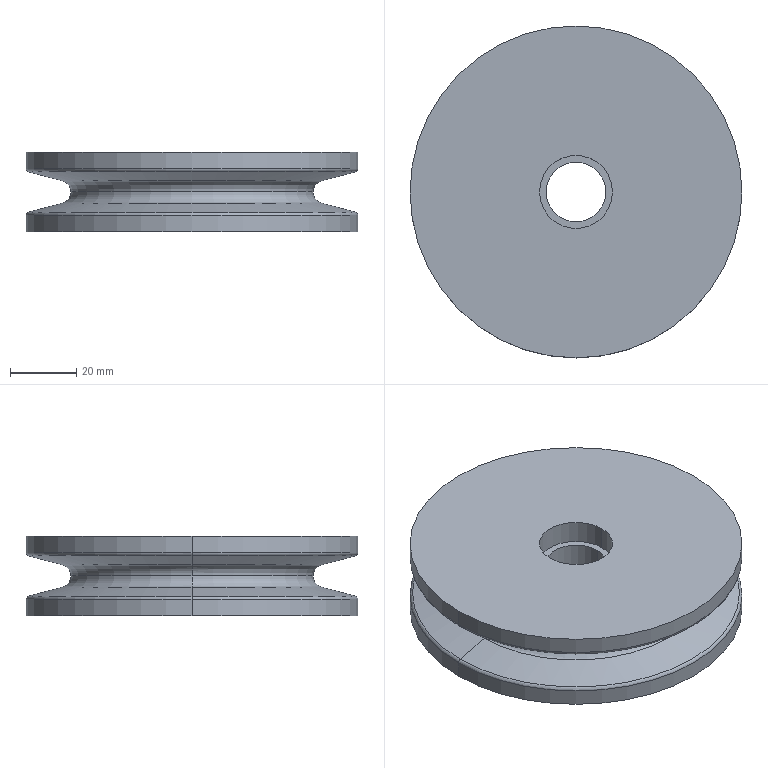Component | SolidWorks | JL001-05-02-1_JL001-05-01-004-2 | 1 solid | 26 faces | box 100 x 100 x 24 mm | volume 147536 mm3 | cylinder 10 | torus 8 | cone 4 | plane 4 | commonest cylinder face diameters 22 x4 100 x4 18 x2
build123d program:
from build123d import *

# Parameters (mm, degrees)
FILLET1_R = 1


with BuildPart() as part:
    # Sketch1 → Revolve1 (revolve)
    with BuildSketch(Plane.XY, mode=Mode.PRIVATE) as revolve1_sk:
        Polygon((11, 12), (50, 12), (50, -12), (11, -12), (11, -5), (9, -5), (9, 5), (11, 5), align=None)
    revolve(revolve1_sk.sketch.rotate(Axis((0, 0, 0), (0, -1, 0)), 90), axis=Axis((0, 0, 0), (0, -1, 0)))

    # Sketch2 → Cut-Revolve1 (revolve, cut)
    with BuildSketch(Plane.XY, mode=Mode.PRIVATE) as cut_revolve1_sk:
        with BuildLine():
            Line((39.094, 3.381), (51, 6.571))
            Line((51, 6.571), (51, -6.571))
            Line((51, -6.571), (39.094, -3.381))
            ThreePointArc((39.094, -3.381), (36.5, 0), (39.094, 3.381))
        make_face()
    revolve(cut_revolve1_sk.sketch.rotate(Axis((0, 0, 0), (0, -1, 0)), 90), axis=Axis((0, 0, 0), (0, -1, 0)), mode=Mode.SUBTRACT)

    # Fillet1
    fillet1_edges = [part.edges().sort_by_distance(p)[0] for p in [
        (0, -6.303, -50),
        (0, 6.303, -50),
    ]]
    fillet(fillet1_edges, radius=FILLET1_R)


solid = part.part

# Placed as in the assembly
solid = solid.moved(Location((0, 1047.5, 76), (90, 0, 0)))
STEP:
#1=COLOUR_RGB('',0.7922,0.8196,0.9333);
#2=FILL_AREA_STYLE_COLOUR('',#1);
#3=FILL_AREA_STYLE('',(#2));
#4=SURFACE_STYLE_FILL_AREA(#3);
#5=SURFACE_SIDE_STYLE('',(#4));
#6=SURFACE_STYLE_USAGE(.BOTH.,#5);
#7=PRESENTATION_STYLE_ASSIGNMENT((#6));
#8=CARTESIAN_POINT('',(-1.539,41.24,2.859));
#9=VERTEX_POINT('',#8);
#10=CARTESIAN_POINT('',(-1.437,41.24,2.992));
#11=VERTEX_POINT('',#10);
#12=CARTESIAN_POINT('',(-1.575,41.24,2.992));
#13=DIRECTION('',(0.,-1.,0.));
#14=DIRECTION('',(0.,0.,-1.));
#15=AXIS2_PLACEMENT_3D('',#12,#13,#14);
#16=CIRCLE('',#15,0.1378);
#17=EDGE_CURVE('',#9,#11,#16,.T.);
#18=ORIENTED_EDGE('',*,*,#17,.T.);
#19=CARTESIAN_POINT('',(1.437,41.24,2.992));
#20=VERTEX_POINT('',#19);
#21=CARTESIAN_POINT('',(-0.,41.24,2.992));
#22=DIRECTION('',(-0.,-0.,-1.));
#23=DIRECTION('',(0.,1.,0.));
#24=AXIS2_PLACEMENT_3D('',#21,#22,#23);
#25=CIRCLE('',#24,1.437);
#26=EDGE_CURVE('',#11,#20,#25,.T.);
#27=ORIENTED_EDGE('',*,*,#26,.T.);
#28=CARTESIAN_POINT('',(1.539,41.24,2.859));
#29=VERTEX_POINT('',#28);
#30=CARTESIAN_POINT('',(1.575,41.24,2.992));
#31=DIRECTION('',(-0.,1.,-0.));
#32=DIRECTION('',(0.,0.,1.));
#33=AXIS2_PLACEMENT_3D('',#30,#31,#32);
#34=CIRCLE('',#33,0.1378);
#35=EDGE_CURVE('',#29,#20,#34,.T.);
#36=ORIENTED_EDGE('',*,*,#35,.F.);
#37=CARTESIAN_POINT('',(-0.,41.24,2.859));
#38=DIRECTION('',(-0.,-0.,-1.));
#39=DIRECTION('',(-1.,0.,0.));
#40=AXIS2_PLACEMENT_3D('',#37,#38,#39);
#41=CIRCLE('',#40,1.539);
#42=EDGE_CURVE('',#9,#29,#41,.T.);
#43=ORIENTED_EDGE('',*,*,#42,.F.);
#44=EDGE_LOOP('',(#18,#27,#36,#43));
#45=FACE_OUTER_BOUND('',#44,.T.);
#46=CARTESIAN_POINT('',(-0.,41.24,2.992));
#47=DIRECTION('',(-0.,-0.,-1.));
#48=DIRECTION('',(-1.,0.,0.));
#49=AXIS2_PLACEMENT_3D('',#46,#47,#48);
#50=TOROIDAL_SURFACE('',#49,1.575,0.1378);
#51=ADVANCED_FACE('',(#45),#50,.F.);
#52=ORIENTED_EDGE('',*,*,#35,.T.);
#53=CARTESIAN_POINT('',(-0.,41.24,2.992));
#54=DIRECTION('',(-0.,-0.,-1.));
#55=DIRECTION('',(0.,1.,0.));
#56=AXIS2_PLACEMENT_3D('',#53,#54,#55);
#57=CIRCLE('',#56,1.437);
#58=EDGE_CURVE('',#20,#11,#57,.T.);
#59=ORIENTED_EDGE('',*,*,#58,.T.);
#60=ORIENTED_EDGE('',*,*,#17,.F.);
#61=CARTESIAN_POINT('',(-0.,41.24,2.859));
#62=DIRECTION('',(-0.,-0.,-1.));
#63=DIRECTION('',(-1.,0.,0.));
#64=AXIS2_PLACEMENT_3D('',#61,#62,#63);
#65=CIRCLE('',#64,1.539);
#66=EDGE_CURVE('',#29,#9,#65,.T.);
#67=ORIENTED_EDGE('',*,*,#66,.F.);
#68=EDGE_LOOP('',(#52,#59,#60,#67));
#69=FACE_OUTER_BOUND('',#68,.T.);
#70=CARTESIAN_POINT('',(-0.,41.24,2.992));
#71=DIRECTION('',(-0.,-0.,-1.));
#72=DIRECTION('',(-1.,0.,0.));
#73=AXIS2_PLACEMENT_3D('',#70,#71,#72);
#74=TOROIDAL_SURFACE('',#73,1.575,0.1378);
#75=ADVANCED_FACE('',(#69),#74,.F.);
#76=CARTESIAN_POINT('',(1.939,41.24,2.752));
#77=VERTEX_POINT('',#76);
#78=CARTESIAN_POINT('',(-1.939,41.24,2.752));
#79=VERTEX_POINT('',#78);
#80=CARTESIAN_POINT('',(-0.,41.24,2.752));
#81=DIRECTION('',(0.,0.,1.));
#82=DIRECTION('',(-1.,0.,0.));
#83=AXIS2_PLACEMENT_3D('',#80,#81,#82);
#84=CIRCLE('',#83,1.939);
#85=EDGE_CURVE('',#77,#79,#84,.T.);
#86=ORIENTED_EDGE('',*,*,#85,.F.);
#87=CARTESIAN_POINT('',(1.969,41.24,2.714));
#88=VERTEX_POINT('',#87);
#89=CARTESIAN_POINT('',(1.929,41.24,2.714));
#90=DIRECTION('',(-0.,1.,-0.));
#91=DIRECTION('',(0.,0.,1.));
#92=AXIS2_PLACEMENT_3D('',#89,#90,#91);
#93=CIRCLE('',#92,0.03937);
#94=EDGE_CURVE('',#77,#88,#93,.T.);
#95=ORIENTED_EDGE('',*,*,#94,.T.);
#96=CARTESIAN_POINT('',(-1.969,41.24,2.714));
#97=VERTEX_POINT('',#96);
#98=CARTESIAN_POINT('',(-0.,41.24,2.714));
#99=DIRECTION('',(-0.,-0.,-1.));
#100=DIRECTION('',(-1.,0.,0.));
#101=AXIS2_PLACEMENT_3D('',#98,#99,#100);
#102=CIRCLE('',#101,1.969);
#103=EDGE_CURVE('',#97,#88,#102,.T.);
#104=ORIENTED_EDGE('',*,*,#103,.F.);
#105=CARTESIAN_POINT('',(-1.929,41.24,2.714));
#106=DIRECTION('',(0.,-1.,0.));
#107=DIRECTION('',(0.,0.,-1.));
#108=AXIS2_PLACEMENT_3D('',#105,#106,#107);
#109=CIRCLE('',#108,0.03937);
#110=EDGE_CURVE('',#79,#97,#109,.T.);
#111=ORIENTED_EDGE('',*,*,#110,.F.);
#112=EDGE_LOOP('',(#86,#95,#104,#111));
#113=FACE_OUTER_BOUND('',#112,.T.);
#114=CARTESIAN_POINT('',(-0.,41.24,2.714));
#115=DIRECTION('',(-0.,-0.,-1.));
#116=DIRECTION('',(-1.,0.,0.));
#117=AXIS2_PLACEMENT_3D('',#114,#115,#116);
#118=TOROIDAL_SURFACE('',#117,1.929,0.03937);
#119=ADVANCED_FACE('',(#113),#118,.T.);
#120=CARTESIAN_POINT('',(-1.939,41.24,3.232));
#121=VERTEX_POINT('',#120);
#122=CARTESIAN_POINT('',(1.939,41.24,3.232));
#123=VERTEX_POINT('',#122);
#124=CARTESIAN_POINT('',(-0.,41.24,3.232));
#125=DIRECTION('',(-0.,-0.,-1.));
#126=DIRECTION('',(1.,0.,0.));
#127=AXIS2_PLACEMENT_3D('',#124,#125,#126);
#128=CIRCLE('',#127,1.939);
#129=EDGE_CURVE('',#121,#123,#128,.T.);
#130=ORIENTED_EDGE('',*,*,#129,.F.);
#131=CARTESIAN_POINT('',(-1.969,41.24,3.27));
#132=VERTEX_POINT('',#131);
#133=CARTESIAN_POINT('',(-1.929,41.24,3.27));
#134=DIRECTION('',(0.,1.,-0.));
#135=DIRECTION('',(0.,0.,1.));
#136=AXIS2_PLACEMENT_3D('',#133,#134,#135);
#137=CIRCLE('',#136,0.03937);
#138=EDGE_CURVE('',#121,#132,#137,.T.);
#139=ORIENTED_EDGE('',*,*,#138,.T.);
#140=CARTESIAN_POINT('',(1.969,41.24,3.27));
#141=VERTEX_POINT('',#140);
#142=CARTESIAN_POINT('',(-0.,41.24,3.27));
#143=DIRECTION('',(0.,0.,1.));
#144=DIRECTION('',(1.,0.,0.));
#145=AXIS2_PLACEMENT_3D('',#142,#143,#144);
#146=CIRCLE('',#145,1.969);
#147=EDGE_CURVE('',#141,#132,#146,.T.);
#148=ORIENTED_EDGE('',*,*,#147,.F.);
#149=CARTESIAN_POINT('',(1.929,41.24,3.27));
#150=DIRECTION('',(0.,-1.,0.));
#151=DIRECTION('',(0.,0.,-1.));
#152=AXIS2_PLACEMENT_3D('',#149,#150,#151);
#153=CIRCLE('',#152,0.03937);
#154=EDGE_CURVE('',#123,#141,#153,.T.);
#155=ORIENTED_EDGE('',*,*,#154,.F.);
#156=EDGE_LOOP('',(#130,#139,#148,#155));
#157=FACE_OUTER_BOUND('',#156,.T.);
#158=CARTESIAN_POINT('',(-0.,41.24,3.27));
#159=DIRECTION('',(0.,0.,1.));
#160=DIRECTION('',(1.,-0.,-0.));
#161=AXIS2_PLACEMENT_3D('',#158,#159,#160);
#162=TOROIDAL_SURFACE('',#161,1.929,0.03937);
#163=ADVANCED_FACE('',(#157),#162,.T.);
#164=ORIENTED_EDGE('',*,*,#58,.F.);
#165=CARTESIAN_POINT('',(1.539,41.24,3.125));
#166=VERTEX_POINT('',#165);
#167=CARTESIAN_POINT('',(1.575,41.24,2.992));
#168=DIRECTION('',(-0.,1.,-0.));
#169=DIRECTION('',(0.,0.,1.));
#170=AXIS2_PLACEMENT_3D('',#167,#168,#169);
#171=CIRCLE('',#170,0.1378);
#172=EDGE_CURVE('',#20,#166,#171,.T.);
#173=ORIENTED_EDGE('',*,*,#172,.T.);
#174=CARTESIAN_POINT('',(-1.539,41.24,3.125));
#175=VERTEX_POINT('',#174);
#176=CARTESIAN_POINT('',(-0.,41.24,3.125));
#177=DIRECTION('',(-0.,-0.,-1.));
#178=DIRECTION('',(-1.,0.,0.));
#179=AXIS2_PLACEMENT_3D('',#176,#177,#178);
#180=CIRCLE('',#179,1.539);
#181=EDGE_CURVE('',#166,#175,#180,.T.);
#182=ORIENTED_EDGE('',*,*,#181,.T.);
#183=CARTESIAN_POINT('',(-1.575,41.24,2.992));
#184=DIRECTION('',(0.,-1.,0.));
#185=DIRECTION('',(0.,0.,-1.));
#186=AXIS2_PLACEMENT_3D('',#183,#184,#185);
#187=CIRCLE('',#186,0.1378);
#188=EDGE_CURVE('',#11,#175,#187,.T.);
#189=ORIENTED_EDGE('',*,*,#188,.F.);
#190=EDGE_LOOP('',(#164,#173,#182,#189));
#191=FACE_OUTER_BOUND('',#190,.T.);
#192=CARTESIAN_POINT('',(-0.,41.24,2.992));
#193=DIRECTION('',(-0.,-0.,-1.));
#194=DIRECTION('',(-1.,0.,0.));
#195=AXIS2_PLACEMENT_3D('',#192,#193,#194);
#196=TOROIDAL_SURFACE('',#195,1.575,0.1378);
#197=ADVANCED_FACE('',(#191),#196,.F.);
#198=ORIENTED_EDGE('',*,*,#42,.T.);
#199=CARTESIAN_POINT('',(2.008,41.24,2.733));
#200=DIRECTION('',(0.9659,0.,-0.2588));
#201=VECTOR('',#200,39.37);
#202=LINE('',#199,#201);
#203=EDGE_CURVE('',#29,#77,#202,.T.);
#204=ORIENTED_EDGE('',*,*,#203,.T.);
#205=ORIENTED_EDGE('',*,*,#85,.T.);
#206=CARTESIAN_POINT('',(-2.008,41.24,2.733));
#207=DIRECTION('',(-0.9659,-0.,-0.2588));
#208=VECTOR('',#207,39.37);
#209=LINE('',#206,#208);
#210=EDGE_CURVE('',#9,#79,#209,.T.);
#211=ORIENTED_EDGE('',*,*,#210,.F.);
#212=EDGE_LOOP('',(#198,#204,#205,#211));
#213=FACE_OUTER_BOUND('',#212,.T.);
#214=CARTESIAN_POINT('',(-0.,41.24,2.733));
#215=DIRECTION('',(-0.,-0.,-1.));
#216=DIRECTION('',(-1.,0.,0.));
#217=AXIS2_PLACEMENT_3D('',#214,#215,#216);
#218=CONICAL_SURFACE('',#217,2.008,1.309);
#219=ADVANCED_FACE('',(#213),#218,.T.);
#220=CARTESIAN_POINT('',(-0.,41.24,3.125));
#221=DIRECTION('',(-0.,-0.,-1.));
#222=DIRECTION('',(-1.,0.,0.));
#223=AXIS2_PLACEMENT_3D('',#220,#221,#222);
#224=CIRCLE('',#223,1.539);
#225=EDGE_CURVE('',#175,#166,#224,.T.);
#226=ORIENTED_EDGE('',*,*,#225,.F.);
#227=CARTESIAN_POINT('',(-1.539,41.24,3.125));
#228=DIRECTION('',(-0.9659,0.,0.2588));
#229=VECTOR('',#228,39.37);
#230=LINE('',#227,#229);
#231=EDGE_CURVE('',#175,#121,#230,.T.);
#232=ORIENTED_EDGE('',*,*,#231,.T.);
#233=ORIENTED_EDGE('',*,*,#129,.T.);
#234=CARTESIAN_POINT('',(1.539,41.24,3.125));
#235=DIRECTION('',(0.9659,0.,0.2588));
#236=VECTOR('',#235,39.37);
#237=LINE('',#234,#236);
#238=EDGE_CURVE('',#166,#123,#237,.T.);
#239=ORIENTED_EDGE('',*,*,#238,.F.);
#240=EDGE_LOOP('',(#226,#232,#233,#239));
#241=FACE_OUTER_BOUND('',#240,.T.);
#242=CARTESIAN_POINT('',(-0.,41.24,3.125));
#243=DIRECTION('',(0.,0.,1.));
#244=DIRECTION('',(1.,0.,0.));
#245=AXIS2_PLACEMENT_3D('',#242,#243,#244);
#246=CONICAL_SURFACE('',#245,1.539,1.309);
#247=ADVANCED_FACE('',(#241),#246,.T.);
#248=CARTESIAN_POINT('',(0.3543,41.24,3.189));
#249=VERTEX_POINT('',#248);
#250=CARTESIAN_POINT('',(-0.3543,41.24,3.189));
#251=VERTEX_POINT('',#250);
#252=CARTESIAN_POINT('',(-0.,41.24,3.189));
#253=DIRECTION('',(-0.,-0.,-1.));
#254=DIRECTION('',(-1.,0.,0.));
#255=AXIS2_PLACEMENT_3D('',#252,#253,#254);
#256=CIRCLE('',#255,0.3543);
#257=EDGE_CURVE('',#249,#251,#256,.T.);
#258=ORIENTED_EDGE('',*,*,#257,.F.);
#259=CARTESIAN_POINT('',(0.3543,41.24,2.795));
#260=VERTEX_POINT('',#259);
#261=CARTESIAN_POINT('',(0.3543,41.24,2.992));
#262=DIRECTION('',(-0.,-0.,-1.));
#263=VECTOR('',#262,39.37);
#264=LINE('',#261,#263);
#265=EDGE_CURVE('',#249,#260,#264,.T.);
#266=ORIENTED_EDGE('',*,*,#265,.T.);
#267=CARTESIAN_POINT('',(-0.3543,41.24,2.795));
#268=VERTEX_POINT('',#267);
#269=CARTESIAN_POINT('',(-0.,41.24,2.795));
#270=DIRECTION('',(-0.,-0.,-1.));
#271=DIRECTION('',(-1.,0.,0.));
#272=AXIS2_PLACEMENT_3D('',#269,#270,#271);
#273=CIRCLE('',#272,0.3543);
#274=EDGE_CURVE('',#260,#268,#273,.T.);
#275=ORIENTED_EDGE('',*,*,#274,.T.);
#276=CARTESIAN_POINT('',(-0.3543,41.24,2.992));
#277=DIRECTION('',(-0.,-0.,-1.));
#278=VECTOR('',#277,39.37);
#279=LINE('',#276,#278);
#280=EDGE_CURVE('',#251,#268,#279,.T.);
#281=ORIENTED_EDGE('',*,*,#280,.F.);
#282=EDGE_LOOP('',(#258,#266,#275,#281));
#283=FACE_OUTER_BOUND('',#282,.T.);
#284=CARTESIAN_POINT('',(-0.,41.24,2.992));
#285=DIRECTION('',(-0.,-0.,-1.));
#286=DIRECTION('',(-1.,0.,0.));
#287=AXIS2_PLACEMENT_3D('',#284,#285,#286);
#288=CYLINDRICAL_SURFACE('',#287,0.3543);
#289=ADVANCED_FACE('',(#283),#288,.F.);
#290=CARTESIAN_POINT('',(0.4331,41.24,3.465));
#291=VERTEX_POINT('',#290);
#292=CARTESIAN_POINT('',(-0.4331,41.24,3.465));
#293=VERTEX_POINT('',#292);
#294=CARTESIAN_POINT('',(-0.,41.24,3.465));
#295=DIRECTION('',(-0.,-0.,-1.));
#296=DIRECTION('',(-1.,0.,0.));
#297=AXIS2_PLACEMENT_3D('',#294,#295,#296);
#298=CIRCLE('',#297,0.4331);
#299=EDGE_CURVE('',#291,#293,#298,.T.);
#300=ORIENTED_EDGE('',*,*,#299,.F.);
#301=CARTESIAN_POINT('',(0.4331,41.24,3.189));
#302=VERTEX_POINT('',#301);
#303=CARTESIAN_POINT('',(0.4331,41.24,2.992));
#304=DIRECTION('',(-0.,-0.,-1.));
#305=VECTOR('',#304,39.37);
#306=LINE('',#303,#305);
#307=EDGE_CURVE('',#291,#302,#306,.T.);
#308=ORIENTED_EDGE('',*,*,#307,.T.);
#309=CARTESIAN_POINT('',(-0.4331,41.24,3.189));
#310=VERTEX_POINT('',#309);
#311=CARTESIAN_POINT('',(-0.,41.24,3.189));
#312=DIRECTION('',(-0.,-0.,-1.));
#313=DIRECTION('',(-1.,0.,0.));
#314=AXIS2_PLACEMENT_3D('',#311,#312,#313);
#315=CIRCLE('',#314,0.4331);
#316=EDGE_CURVE('',#302,#310,#315,.T.);
#317=ORIENTED_EDGE('',*,*,#316,.T.);
#318=CARTESIAN_POINT('',(-0.4331,41.24,2.992));
#319=DIRECTION('',(-0.,-0.,-1.));
#320=VECTOR('',#319,39.37);
#321=LINE('',#318,#320);
#322=EDGE_CURVE('',#293,#310,#321,.T.);
#323=ORIENTED_EDGE('',*,*,#322,.F.);
#324=EDGE_LOOP('',(#300,#308,#317,#323));
#325=FACE_OUTER_BOUND('',#324,.T.);
#326=CARTESIAN_POINT('',(-0.,41.24,2.992));
#327=DIRECTION('',(-0.,-0.,-1.));
#328=DIRECTION('',(-1.,0.,0.));
#329=AXIS2_PLACEMENT_3D('',#326,#327,#328);
#330=CYLINDRICAL_SURFACE('',#329,0.4331);
#331=ADVANCED_FACE('',(#325),#330,.F.);
#332=CARTESIAN_POINT('',(0.4331,41.24,2.795));
#333=VERTEX_POINT('',#332);
#334=CARTESIAN_POINT('',(-0.4331,41.24,2.795));
#335=VERTEX_POINT('',#334);
#336=CARTESIAN_POINT('',(-0.,41.24,2.795));
#337=DIRECTION('',(-0.,-0.,-1.));
#338=DIRECTION('',(-1.,0.,0.));
#339=AXIS2_PLACEMENT_3D('',#336,#337,#338);
#340=CIRCLE('',#339,0.4331);
#341=EDGE_CURVE('',#333,#335,#340,.T.);
#342=ORIENTED_EDGE('',*,*,#341,.F.);
#343=CARTESIAN_POINT('',(0.4331,41.24,2.52));
#344=VERTEX_POINT('',#343);
#345=CARTESIAN_POINT('',(0.4331,41.24,2.992));
#346=DIRECTION('',(-0.,-0.,-1.));
#347=VECTOR('',#346,39.37);
#348=LINE('',#345,#347);
#349=EDGE_CURVE('',#333,#344,#348,.T.);
#350=ORIENTED_EDGE('',*,*,#349,.T.);
#351=CARTESIAN_POINT('',(-0.4331,41.24,2.52));
#352=VERTEX_POINT('',#351);
#353=CARTESIAN_POINT('',(-0.,41.24,2.52));
#354=DIRECTION('',(-0.,-0.,-1.));
#355=DIRECTION('',(-1.,0.,0.));
#356=AXIS2_PLACEMENT_3D('',#353,#354,#355);
#357=CIRCLE('',#356,0.4331);
#358=EDGE_CURVE('',#344,#352,#357,.T.);
#359=ORIENTED_EDGE('',*,*,#358,.T.);
#360=CARTESIAN_POINT('',(-0.4331,41.24,2.992));
#361=DIRECTION('',(-0.,-0.,-1.));
#362=VECTOR('',#361,39.37);
#363=LINE('',#360,#362);
#364=EDGE_CURVE('',#335,#352,#363,.T.);
#365=ORIENTED_EDGE('',*,*,#364,.F.);
#366=EDGE_LOOP('',(#342,#350,#359,#365));
#367=FACE_OUTER_BOUND('',#366,.T.);
#368=CARTESIAN_POINT('',(-0.,41.24,2.992));
#369=DIRECTION('',(-0.,-0.,-1.));
#370=DIRECTION('',(-1.,0.,0.));
#371=AXIS2_PLACEMENT_3D('',#368,#369,#370);
#372=CYLINDRICAL_SURFACE('',#371,0.4331);
#373=ADVANCED_FACE('',(#367),#372,.F.);
#374=ORIENTED_EDGE('',*,*,#103,.T.);
#375=CARTESIAN_POINT('',(1.969,41.24,2.52));
#376=VERTEX_POINT('',#375);
#377=CARTESIAN_POINT('',(1.969,41.24,2.992));
#378=DIRECTION('',(-0.,-0.,-1.));
#379=VECTOR('',#378,39.37);
#380=LINE('',#377,#379);
#381=EDGE_CURVE('',#88,#376,#380,.T.);
#382=ORIENTED_EDGE('',*,*,#381,.T.);
#383=CARTESIAN_POINT('',(-1.969,41.24,2.52));
#384=VERTEX_POINT('',#383);
#385=CARTESIAN_POINT('',(-0.,41.24,2.52));
#386=DIRECTION('',(-0.,-0.,-1.));
#387=DIRECTION('',(-1.,0.,0.));
#388=AXIS2_PLACEMENT_3D('',#385,#386,#387);
#389=CIRCLE('',#388,1.969);
#390=EDGE_CURVE('',#384,#376,#389,.T.);
#391=ORIENTED_EDGE('',*,*,#390,.F.);
#392=CARTESIAN_POINT('',(-1.969,41.24,2.992));
#393=DIRECTION('',(-0.,-0.,-1.));
#394=VECTOR('',#393,39.37);
#395=LINE('',#392,#394);
#396=EDGE_CURVE('',#97,#384,#395,.T.);
#397=ORIENTED_EDGE('',*,*,#396,.F.);
#398=EDGE_LOOP('',(#374,#382,#391,#397));
#399=FACE_OUTER_BOUND('',#398,.T.);
#400=CARTESIAN_POINT('',(-0.,41.24,2.992));
#401=DIRECTION('',(-0.,-0.,-1.));
#402=DIRECTION('',(-1.,0.,0.));
#403=AXIS2_PLACEMENT_3D('',#400,#401,#402);
#404=CYLINDRICAL_SURFACE('',#403,1.969);
#405=ADVANCED_FACE('',(#399),#404,.T.);
#406=CARTESIAN_POINT('',(-1.969,41.24,3.465));
#407=VERTEX_POINT('',#406);
#408=CARTESIAN_POINT('',(1.969,41.24,3.465));
#409=VERTEX_POINT('',#408);
#410=CARTESIAN_POINT('',(-0.,41.24,3.465));
#411=DIRECTION('',(-0.,-0.,-1.));
#412=DIRECTION('',(-1.,0.,0.));
#413=AXIS2_PLACEMENT_3D('',#410,#411,#412);
#414=CIRCLE('',#413,1.969);
#415=EDGE_CURVE('',#407,#409,#414,.T.);
#416=ORIENTED_EDGE('',*,*,#415,.T.);
#417=CARTESIAN_POINT('',(1.969,41.24,2.992));
#418=DIRECTION('',(-0.,-0.,-1.));
#419=VECTOR('',#418,39.37);
#420=LINE('',#417,#419);
#421=EDGE_CURVE('',#409,#141,#420,.T.);
#422=ORIENTED_EDGE('',*,*,#421,.T.);
#423=ORIENTED_EDGE('',*,*,#147,.T.);
#424=CARTESIAN_POINT('',(-1.969,41.24,2.992));
#425=DIRECTION('',(-0.,-0.,-1.));
#426=VECTOR('',#425,39.37);
#427=LINE('',#424,#426);
#428=EDGE_CURVE('',#407,#132,#427,.T.);
#429=ORIENTED_EDGE('',*,*,#428,.F.);
#430=EDGE_LOOP('',(#416,#422,#423,#429));
#431=FACE_OUTER_BOUND('',#430,.T.);
#432=CARTESIAN_POINT('',(-0.,41.24,2.992));
#433=DIRECTION('',(-0.,-0.,-1.));
#434=DIRECTION('',(-1.,0.,0.));
#435=AXIS2_PLACEMENT_3D('',#432,#433,#434);
#436=CYLINDRICAL_SURFACE('',#435,1.969);
#437=ADVANCED_FACE('',(#431),#436,.T.);
#438=ORIENTED_EDGE('',*,*,#421,.F.);
#439=CARTESIAN_POINT('',(-0.,41.24,3.465));
#440=DIRECTION('',(-0.,-0.,-1.));
#441=DIRECTION('',(-1.,0.,0.));
#442=AXIS2_PLACEMENT_3D('',#439,#440,#441);
#443=CIRCLE('',#442,1.969);
#444=EDGE_CURVE('',#409,#407,#443,.T.);
#445=ORIENTED_EDGE('',*,*,#444,.T.);
#446=ORIENTED_EDGE('',*,*,#428,.T.);
#447=CARTESIAN_POINT('',(-0.,41.24,3.27));
#448=DIRECTION('',(0.,0.,1.));
#449=DIRECTION('',(1.,0.,0.));
#450=AXIS2_PLACEMENT_3D('',#447,#448,#449);
#451=CIRCLE('',#450,1.969);
#452=EDGE_CURVE('',#132,#141,#451,.T.);
#453=ORIENTED_EDGE('',*,*,#452,.T.);
#454=EDGE_LOOP('',(#438,#445,#446,#453));
#455=FACE_OUTER_BOUND('',#454,.T.);
#456=CARTESIAN_POINT('',(-0.,41.24,2.992));
#457=DIRECTION('',(-0.,-0.,-1.));
#458=DIRECTION('',(-1.,0.,0.));
#459=AXIS2_PLACEMENT_3D('',#456,#457,#458);
#460=CYLINDRICAL_SURFACE('',#459,1.969);
#461=ADVANCED_FACE('',(#455),#460,.T.);
#462=ORIENTED_EDGE('',*,*,#381,.F.);
#463=CARTESIAN_POINT('',(-0.,41.24,2.714));
#464=DIRECTION('',(-0.,-0.,-1.));
#465=DIRECTION('',(-1.,0.,0.));
#466=AXIS2_PLACEMENT_3D('',#463,#464,#465);
#467=CIRCLE('',#466,1.969);
#468=EDGE_CURVE('',#88,#97,#467,.T.);
#469=ORIENTED_EDGE('',*,*,#468,.T.);
#470=ORIENTED_EDGE('',*,*,#396,.T.);
#471=CARTESIAN_POINT('',(-0.,41.24,2.52));
#472=DIRECTION('',(-0.,-0.,-1.));
#473=DIRECTION('',(-1.,0.,0.));
#474=AXIS2_PLACEMENT_3D('',#471,#472,#473);
#475=CIRCLE('',#474,1.969);
#476=EDGE_CURVE('',#376,#384,#475,.T.);
#477=ORIENTED_EDGE('',*,*,#476,.F.);
#478=EDGE_LOOP('',(#462,#469,#470,#477));
#479=FACE_OUTER_BOUND('',#478,.T.);
#480=CARTESIAN_POINT('',(-0.,41.24,2.992));
#481=DIRECTION('',(-0.,-0.,-1.));
#482=DIRECTION('',(-1.,0.,0.));
#483=AXIS2_PLACEMENT_3D('',#480,#481,#482);
#484=CYLINDRICAL_SURFACE('',#483,1.969);
#485=ADVANCED_FACE('',(#479),#484,.T.);
#486=ORIENTED_EDGE('',*,*,#349,.F.);
#487=CARTESIAN_POINT('',(-0.,41.24,2.795));
#488=DIRECTION('',(-0.,-0.,-1.));
#489=DIRECTION('',(-1.,0.,0.));
#490=AXIS2_PLACEMENT_3D('',#487,#488,#489);
#491=CIRCLE('',#490,0.4331);
#492=EDGE_CURVE('',#335,#333,#491,.T.);
#493=ORIENTED_EDGE('',*,*,#492,.F.);
#494=ORIENTED_EDGE('',*,*,#364,.T.);
#495=CARTESIAN_POINT('',(-0.,41.24,2.52));
#496=DIRECTION('',(-0.,-0.,-1.));
#497=DIRECTION('',(-1.,0.,0.));
#498=AXIS2_PLACEMENT_3D('',#495,#496,#497);
#499=CIRCLE('',#498,0.4331);
#500=EDGE_CURVE('',#352,#344,#499,.T.);
#501=ORIENTED_EDGE('',*,*,#500,.T.);
#502=EDGE_LOOP('',(#486,#493,#494,#501));
#503=FACE_OUTER_BOUND('',#502,.T.);
#504=CARTESIAN_POINT('',(-0.,41.24,2.992));
#505=DIRECTION('',(-0.,-0.,-1.));
#506=DIRECTION('',(-1.,0.,0.));
#507=AXIS2_PLACEMENT_3D('',#504,#505,#506);
#508=CYLINDRICAL_SURFACE('',#507,0.4331);
#509=ADVANCED_FACE('',(#503),#508,.F.);
#510=ORIENTED_EDGE('',*,*,#500,.F.);
#511=ORIENTED_EDGE('',*,*,#358,.F.);
#512=EDGE_LOOP('',(#510,#511));
#513=FACE_BOUND('',#512,.T.);
#514=ORIENTED_EDGE('',*,*,#390,.T.);
#515=ORIENTED_EDGE('',*,*,#476,.T.);
#516=EDGE_LOOP('',(#514,#515));
#517=FACE_OUTER_BOUND('',#516,.T.);
#518=CARTESIAN_POINT('',(-0.,41.673,2.52));
#519=DIRECTION('',(0.,0.,1.));
#520=DIRECTION('',(1.,0.,-0.));
#521=AXIS2_PLACEMENT_3D('',#518,#519,#520);
#522=PLANE('',#521);
#523=ADVANCED_FACE('',(#513,#517),#522,.F.);
#524=ORIENTED_EDGE('',*,*,#415,.F.);
#525=ORIENTED_EDGE('',*,*,#444,.F.);
#526=EDGE_LOOP('',(#524,#525));
#527=FACE_OUTER_BOUND('',#526,.T.);
#528=CARTESIAN_POINT('',(-0.,41.24,3.465));
#529=DIRECTION('',(-0.,-0.,-1.));
#530=DIRECTION('',(-1.,0.,0.));
#531=AXIS2_PLACEMENT_3D('',#528,#529,#530);
#532=CIRCLE('',#531,0.4331);
#533=EDGE_CURVE('',#293,#291,#532,.T.);
#534=ORIENTED_EDGE('',*,*,#533,.T.);
#535=ORIENTED_EDGE('',*,*,#299,.T.);
#536=EDGE_LOOP('',(#534,#535));
#537=FACE_BOUND('',#536,.T.);
#538=CARTESIAN_POINT('',(-0.,43.209,3.465));
#539=DIRECTION('',(-0.,-0.,-1.));
#540=DIRECTION('',(-1.,0.,0.));
#541=AXIS2_PLACEMENT_3D('',#538,#539,#540);
#542=PLANE('',#541);
#543=ADVANCED_FACE('',(#527,#537),#542,.F.);
#544=ORIENTED_EDGE('',*,*,#307,.F.);
#545=ORIENTED_EDGE('',*,*,#533,.F.);
#546=ORIENTED_EDGE('',*,*,#322,.T.);
#547=CARTESIAN_POINT('',(-0.,41.24,3.189));
#548=DIRECTION('',(-0.,-0.,-1.));
#549=DIRECTION('',(-1.,0.,0.));
#550=AXIS2_PLACEMENT_3D('',#547,#548,#549);
#551=CIRCLE('',#550,0.4331);
#552=EDGE_CURVE('',#310,#302,#551,.T.);
#553=ORIENTED_EDGE('',*,*,#552,.T.);
#554=EDGE_LOOP('',(#544,#545,#546,#553));
#555=FACE_OUTER_BOUND('',#554,.T.);
#556=CARTESIAN_POINT('',(-0.,41.24,2.992));
#557=DIRECTION('',(-0.,-0.,-1.));
#558=DIRECTION('',(-1.,0.,0.));
#559=AXIS2_PLACEMENT_3D('',#556,#557,#558);
#560=CYLINDRICAL_SURFACE('',#559,0.4331);
#561=ADVANCED_FACE('',(#555),#560,.F.);
#562=ORIENTED_EDGE('',*,*,#552,.F.);
#563=ORIENTED_EDGE('',*,*,#316,.F.);
#564=EDGE_LOOP('',(#562,#563));
#565=FACE_OUTER_BOUND('',#564,.T.);
#566=CARTESIAN_POINT('',(-0.,41.24,3.189));
#567=DIRECTION('',(-0.,-0.,-1.));
#568=DIRECTION('',(-1.,0.,0.));
#569=AXIS2_PLACEMENT_3D('',#566,#567,#568);
#570=CIRCLE('',#569,0.3543);
#571=EDGE_CURVE('',#251,#249,#570,.T.);
#572=ORIENTED_EDGE('',*,*,#571,.T.);
#573=ORIENTED_EDGE('',*,*,#257,.T.);
#574=EDGE_LOOP('',(#572,#573));
#575=FACE_BOUND('',#574,.T.);
#576=CARTESIAN_POINT('',(-0.,41.673,3.189));
#577=DIRECTION('',(-0.,-0.,-1.));
#578=DIRECTION('',(-1.,0.,0.));
#579=AXIS2_PLACEMENT_3D('',#576,#577,#578);
#580=PLANE('',#579);
#581=ADVANCED_FACE('',(#565,#575),#580,.F.);
#582=ORIENTED_EDGE('',*,*,#265,.F.);
#583=ORIENTED_EDGE('',*,*,#571,.F.);
#584=ORIENTED_EDGE('',*,*,#280,.T.);
#585=CARTESIAN_POINT('',(-0.,41.24,2.795));
#586=DIRECTION('',(-0.,-0.,-1.));
#587=DIRECTION('',(-1.,0.,0.));
#588=AXIS2_PLACEMENT_3D('',#585,#586,#587);
#589=CIRCLE('',#588,0.3543);
#590=EDGE_CURVE('',#268,#260,#589,.T.);
#591=ORIENTED_EDGE('',*,*,#590,.T.);
#592=EDGE_LOOP('',(#582,#583,#584,#591));
#593=FACE_OUTER_BOUND('',#592,.T.);
#594=CARTESIAN_POINT('',(-0.,41.24,2.992));
#595=DIRECTION('',(-0.,-0.,-1.));
#596=DIRECTION('',(-1.,0.,0.));
#597=AXIS2_PLACEMENT_3D('',#594,#595,#596);
#598=CYLINDRICAL_SURFACE('',#597,0.3543);
#599=ADVANCED_FACE('',(#593),#598,.F.);
#600=ORIENTED_EDGE('',*,*,#590,.F.);
#601=ORIENTED_EDGE('',*,*,#274,.F.);
#602=EDGE_LOOP('',(#600,#601));
#603=FACE_BOUND('',#602,.T.);
#604=ORIENTED_EDGE('',*,*,#492,.T.);
#605=ORIENTED_EDGE('',*,*,#341,.T.);
#606=EDGE_LOOP('',(#604,#605));
#607=FACE_OUTER_BOUND('',#606,.T.);
#608=CARTESIAN_POINT('',(-0.,41.594,2.795));
#609=DIRECTION('',(0.,0.,1.));
#610=DIRECTION('',(1.,0.,-0.));
#611=AXIS2_PLACEMENT_3D('',#608,#609,#610);
#612=PLANE('',#611);
#613=ADVANCED_FACE('',(#603,#607),#612,.F.);
#614=ORIENTED_EDGE('',*,*,#231,.F.);
#615=ORIENTED_EDGE('',*,*,#181,.F.);
#616=ORIENTED_EDGE('',*,*,#238,.T.);
#617=CARTESIAN_POINT('',(-0.,41.24,3.232));
#618=DIRECTION('',(-0.,-0.,-1.));
#619=DIRECTION('',(1.,0.,0.));
#620=AXIS2_PLACEMENT_3D('',#617,#618,#619);
#621=CIRCLE('',#620,1.939);
#622=EDGE_CURVE('',#123,#121,#621,.T.);
#623=ORIENTED_EDGE('',*,*,#622,.T.);
#624=EDGE_LOOP('',(#614,#615,#616,#623));
#625=FACE_OUTER_BOUND('',#624,.T.);
#626=CARTESIAN_POINT('',(-0.,41.24,3.125));
#627=DIRECTION('',(0.,0.,1.));
#628=DIRECTION('',(1.,0.,0.));
#629=AXIS2_PLACEMENT_3D('',#626,#627,#628);
#630=CONICAL_SURFACE('',#629,1.539,1.309);
#631=ADVANCED_FACE('',(#625),#630,.T.);
#632=ORIENTED_EDGE('',*,*,#203,.F.);
#633=ORIENTED_EDGE('',*,*,#66,.T.);
#634=ORIENTED_EDGE('',*,*,#210,.T.);
#635=CARTESIAN_POINT('',(-0.,41.24,2.752));
#636=DIRECTION('',(0.,0.,1.));
#637=DIRECTION('',(-1.,0.,0.));
#638=AXIS2_PLACEMENT_3D('',#635,#636,#637);
#639=CIRCLE('',#638,1.939);
#640=EDGE_CURVE('',#79,#77,#639,.T.);
#641=ORIENTED_EDGE('',*,*,#640,.T.);
#642=EDGE_LOOP('',(#632,#633,#634,#641));
#643=FACE_OUTER_BOUND('',#642,.T.);
#644=CARTESIAN_POINT('',(-0.,41.24,2.733));
#645=DIRECTION('',(-0.,-0.,-1.));
#646=DIRECTION('',(-1.,0.,0.));
#647=AXIS2_PLACEMENT_3D('',#644,#645,#646);
#648=CONICAL_SURFACE('',#647,2.008,1.309);
#649=ADVANCED_FACE('',(#643),#648,.T.);
#650=ORIENTED_EDGE('',*,*,#26,.F.);
#651=ORIENTED_EDGE('',*,*,#188,.T.);
#652=ORIENTED_EDGE('',*,*,#225,.T.);
#653=ORIENTED_EDGE('',*,*,#172,.F.);
#654=EDGE_LOOP('',(#650,#651,#652,#653));
#655=FACE_OUTER_BOUND('',#654,.T.);
#656=CARTESIAN_POINT('',(-0.,41.24,2.992));
#657=DIRECTION('',(-0.,-0.,-1.));
#658=DIRECTION('',(-1.,0.,0.));
#659=AXIS2_PLACEMENT_3D('',#656,#657,#658);
#660=TOROIDAL_SURFACE('',#659,1.575,0.1378);
#661=ADVANCED_FACE('',(#655),#660,.F.);
#662=ORIENTED_EDGE('',*,*,#138,.F.);
#663=ORIENTED_EDGE('',*,*,#622,.F.);
#664=ORIENTED_EDGE('',*,*,#154,.T.);
#665=ORIENTED_EDGE('',*,*,#452,.F.);
#666=EDGE_LOOP('',(#662,#663,#664,#665));
#667=FACE_OUTER_BOUND('',#666,.T.);
#668=CARTESIAN_POINT('',(-0.,41.24,3.27));
#669=DIRECTION('',(0.,0.,1.));
#670=DIRECTION('',(1.,-0.,-0.));
#671=AXIS2_PLACEMENT_3D('',#668,#669,#670);
#672=TOROIDAL_SURFACE('',#671,1.929,0.03937);
#673=ADVANCED_FACE('',(#667),#672,.T.);
#674=ORIENTED_EDGE('',*,*,#94,.F.);
#675=ORIENTED_EDGE('',*,*,#640,.F.);
#676=ORIENTED_EDGE('',*,*,#110,.T.);
#677=ORIENTED_EDGE('',*,*,#468,.F.);
#678=EDGE_LOOP('',(#674,#675,#676,#677));
#679=FACE_OUTER_BOUND('',#678,.T.);
#680=CARTESIAN_POINT('',(-0.,41.24,2.714));
#681=DIRECTION('',(-0.,-0.,-1.));
#682=DIRECTION('',(-1.,0.,0.));
#683=AXIS2_PLACEMENT_3D('',#680,#681,#682);
#684=TOROIDAL_SURFACE('',#683,1.929,0.03937);
#685=ADVANCED_FACE('',(#679),#684,.T.);
#686=CLOSED_SHELL('',(#51,#75,#119,#163,#197,#219,#247,#289,#331,#373,#405,#437,#461,#485,#509,#523,#543,#561,#581,#599,#613,#631,#649,#661,#673,#685));
#687=MANIFOLD_SOLID_BREP('',#686);
#688=STYLED_ITEM('',(#7),#687);
#689=(LENGTH_UNIT()NAMED_UNIT(*)SI_UNIT($,.METRE.));
#690=LENGTH_MEASURE_WITH_UNIT(LENGTH_MEASURE(0.0254),#689);
#691=DIMENSIONAL_EXPONENTS(1.,0.,0.,0.,0.,0.,0.);
#692=(CONVERSION_BASED_UNIT('',#690)LENGTH_UNIT()NAMED_UNIT(#691));
#693=UNCERTAINTY_MEASURE_WITH_UNIT(LENGTH_MEASURE(0.00001),#692,'','');
#694=(NAMED_UNIT(*)PLANE_ANGLE_UNIT()SI_UNIT($,.RADIAN.));
#695=(NAMED_UNIT(*)SI_UNIT($,.STERADIAN.)SOLID_ANGLE_UNIT());
#696=(GEOMETRIC_REPRESENTATION_CONTEXT(3)GLOBAL_UNCERTAINTY_ASSIGNED_CONTEXT((#693))GLOBAL_UNIT_ASSIGNED_CONTEXT((#692,#694,#695))REPRESENTATION_CONTEXT('',''));
#697=MECHANICAL_DESIGN_GEOMETRIC_PRESENTATION_REPRESENTATION('',(#688),#696);
#698=CARTESIAN_POINT('',(0.,0.,0.));
#699=DIRECTION('',(0.,0.,1.));
#700=DIRECTION('',(1.,0.,0.));
#701=AXIS2_PLACEMENT_3D('',#698,#699,#700);
#702=(LENGTH_UNIT()NAMED_UNIT(*)SI_UNIT($,.METRE.));
#703=LENGTH_MEASURE_WITH_UNIT(LENGTH_MEASURE(0.0254),#702);
#704=DIMENSIONAL_EXPONENTS(1.,0.,0.,0.,0.,0.,0.);
#705=(CONVERSION_BASED_UNIT('',#703)LENGTH_UNIT()NAMED_UNIT(#704));
#706=UNCERTAINTY_MEASURE_WITH_UNIT(LENGTH_MEASURE(0.00001),#705,'','');
#707=(NAMED_UNIT(*)PLANE_ANGLE_UNIT()SI_UNIT($,.RADIAN.));
#708=(NAMED_UNIT(*)SI_UNIT($,.STERADIAN.)SOLID_ANGLE_UNIT());
#709=(GEOMETRIC_REPRESENTATION_CONTEXT(3)GLOBAL_UNCERTAINTY_ASSIGNED_CONTEXT((#706))GLOBAL_UNIT_ASSIGNED_CONTEXT((#705,#707,#708))REPRESENTATION_CONTEXT('',''));
#710=ADVANCED_BREP_SHAPE_REPRESENTATION('',(#687,#701),#709);
#711=PRESENTATION_LAYER_ASSIGNMENT('','',(#688));